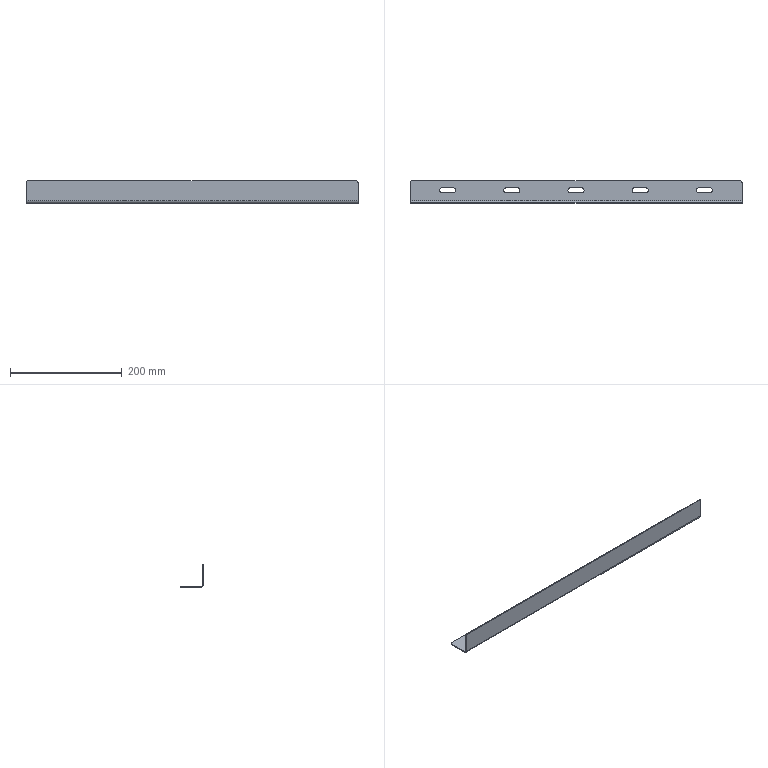Component | SolidWorks | FrameLongitudinalBeamThree40001100-3 | 1 solid | 38 faces | volume 66978 mm3 | plane 22 | cylinder 16 | commonest cylinder face diameters 9 x10 6 x4 8 x1 5 x1